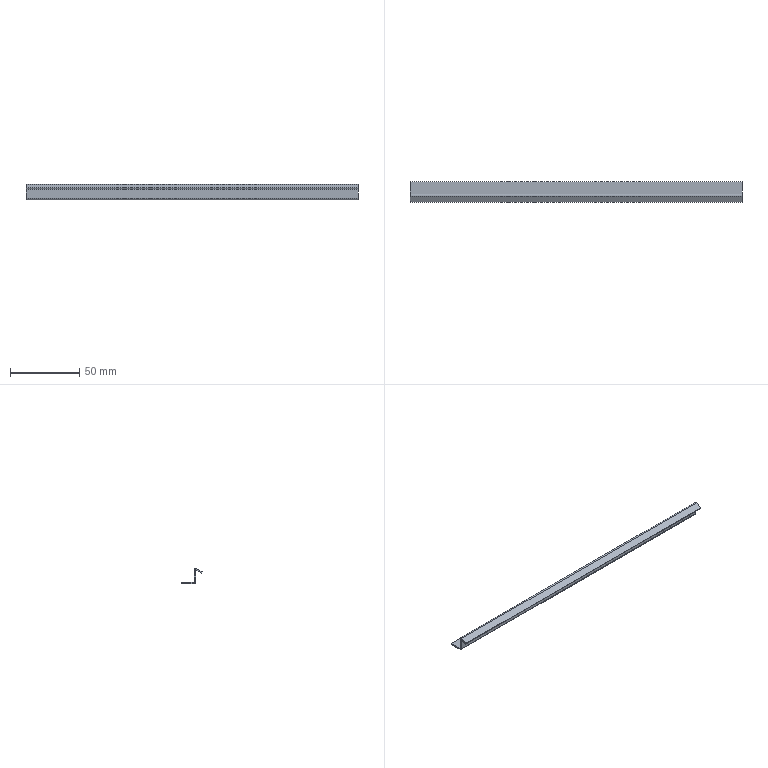Component | SolidWorks | Lampshade-1_Lampshade4-2 | 1 solid | 22 faces | box 240 x 14.83 x 10.93 mm | volume 5917 mm3 | plane 18 | cylinder 4 | commonest cylinder face diameters 2.2 x2 0.2 x2
STEP:
#1=COLOUR_RGB('',0.7922,0.8196,0.9333);
#2=FILL_AREA_STYLE_COLOUR('',#1);
#3=FILL_AREA_STYLE('',(#2));
#4=SURFACE_STYLE_FILL_AREA(#3);
#5=SURFACE_SIDE_STYLE('',(#4));
#6=SURFACE_STYLE_USAGE(.BOTH.,#5);
#7=PRESENTATION_STYLE_ASSIGNMENT((#6));
#8=CARTESIAN_POINT('',(-6.077,-0.7475,2.165));
#9=VERTEX_POINT('',#8);
#10=CARTESIAN_POINT('',(-6.077,-0.7475,2.205));
#11=VERTEX_POINT('',#10);
#12=CARTESIAN_POINT('',(-6.077,-0.7475,2.165));
#13=DIRECTION('',(-0.,0.,1.));
#14=VECTOR('',#13,39.37);
#15=LINE('',#12,#14);
#16=EDGE_CURVE('',#9,#11,#15,.T.);
#17=ORIENTED_EDGE('',*,*,#16,.F.);
#18=CARTESIAN_POINT('',(-6.077,-0.7908,2.209));
#19=VERTEX_POINT('',#18);
#20=CARTESIAN_POINT('',(-6.077,-0.7475,2.209));
#21=DIRECTION('',(-1.,0.,-0.));
#22=DIRECTION('',(0.,0.,-1.));
#23=AXIS2_PLACEMENT_3D('',#20,#21,#22);
#24=CIRCLE('',#23,0.04331);
#25=EDGE_CURVE('',#9,#19,#24,.T.);
#26=ORIENTED_EDGE('',*,*,#25,.T.);
#27=CARTESIAN_POINT('',(-6.077,-0.7514,2.209));
#28=VERTEX_POINT('',#27);
#29=CARTESIAN_POINT('',(-6.077,-0.7514,2.209));
#30=DIRECTION('',(-0.,-1.,0.));
#31=VECTOR('',#30,39.37);
#32=LINE('',#29,#31);
#33=EDGE_CURVE('',#28,#19,#32,.T.);
#34=ORIENTED_EDGE('',*,*,#33,.F.);
#35=CARTESIAN_POINT('',(-6.077,-0.7475,2.209));
#36=DIRECTION('',(-1.,0.,-0.));
#37=DIRECTION('',(0.,0.,1.));
#38=AXIS2_PLACEMENT_3D('',#35,#36,#37);
#39=CIRCLE('',#38,0.003937);
#40=EDGE_CURVE('',#11,#28,#39,.T.);
#41=ORIENTED_EDGE('',*,*,#40,.F.);
#42=EDGE_LOOP('',(#17,#26,#34,#41));
#43=FACE_OUTER_BOUND('',#42,.T.);
#44=CARTESIAN_POINT('',(-6.077,-0.7475,2.165));
#45=DIRECTION('',(-1.,0.,-0.));
#46=DIRECTION('',(-0.,0.,1.));
#47=AXIS2_PLACEMENT_3D('',#44,#45,#46);
#48=PLANE('',#47);
#49=ADVANCED_FACE('',(#43),#48,.T.);
#50=CARTESIAN_POINT('',(-6.077,-0.3971,2.165));
#51=VERTEX_POINT('',#50);
#52=CARTESIAN_POINT('',(-6.077,-0.3971,2.165));
#53=DIRECTION('',(-0.,-1.,0.));
#54=VECTOR('',#53,39.37);
#55=LINE('',#52,#54);
#56=EDGE_CURVE('',#51,#9,#55,.T.);
#57=ORIENTED_EDGE('',*,*,#56,.T.);
#58=ORIENTED_EDGE('',*,*,#16,.T.);
#59=CARTESIAN_POINT('',(-6.077,-0.3971,2.205));
#60=VERTEX_POINT('',#59);
#61=CARTESIAN_POINT('',(-6.077,-0.3971,2.205));
#62=DIRECTION('',(-0.,-1.,0.));
#63=VECTOR('',#62,39.37);
#64=LINE('',#61,#63);
#65=EDGE_CURVE('',#60,#11,#64,.T.);
#66=ORIENTED_EDGE('',*,*,#65,.F.);
#67=CARTESIAN_POINT('',(-6.077,-0.3971,2.165));
#68=DIRECTION('',(-0.,0.,1.));
#69=VECTOR('',#68,39.37);
#70=LINE('',#67,#69);
#71=EDGE_CURVE('',#51,#60,#70,.T.);
#72=ORIENTED_EDGE('',*,*,#71,.F.);
#73=EDGE_LOOP('',(#57,#58,#66,#72));
#74=FACE_OUTER_BOUND('',#73,.T.);
#75=CARTESIAN_POINT('',(-6.077,-0.7514,2.209));
#76=DIRECTION('',(-1.,0.,-0.));
#77=DIRECTION('',(-0.,0.,1.));
#78=AXIS2_PLACEMENT_3D('',#75,#76,#77);
#79=PLANE('',#78);
#80=ADVANCED_FACE('',(#74),#79,.T.);
#81=CARTESIAN_POINT('',(3.372,-0.7908,2.209));
#82=VERTEX_POINT('',#81);
#83=CARTESIAN_POINT('',(3.372,-0.7514,2.209));
#84=VERTEX_POINT('',#83);
#85=CARTESIAN_POINT('',(3.372,-0.7908,2.209));
#86=DIRECTION('',(0.,1.,-0.));
#87=VECTOR('',#86,39.37);
#88=LINE('',#85,#87);
#89=EDGE_CURVE('',#82,#84,#88,.T.);
#90=ORIENTED_EDGE('',*,*,#89,.F.);
#91=CARTESIAN_POINT('',(3.372,-0.7475,2.165));
#92=VERTEX_POINT('',#91);
#93=CARTESIAN_POINT('',(3.372,-0.7475,2.209));
#94=DIRECTION('',(-1.,0.,-0.));
#95=DIRECTION('',(0.,0.,-1.));
#96=AXIS2_PLACEMENT_3D('',#93,#94,#95);
#97=CIRCLE('',#96,0.04331);
#98=EDGE_CURVE('',#92,#82,#97,.T.);
#99=ORIENTED_EDGE('',*,*,#98,.F.);
#100=CARTESIAN_POINT('',(3.372,-0.7475,2.205));
#101=VERTEX_POINT('',#100);
#102=CARTESIAN_POINT('',(3.372,-0.7475,2.205));
#103=DIRECTION('',(0.,-0.,-1.));
#104=VECTOR('',#103,39.37);
#105=LINE('',#102,#104);
#106=EDGE_CURVE('',#101,#92,#105,.T.);
#107=ORIENTED_EDGE('',*,*,#106,.F.);
#108=CARTESIAN_POINT('',(3.372,-0.7475,2.209));
#109=DIRECTION('',(-1.,0.,-0.));
#110=DIRECTION('',(0.,0.,1.));
#111=AXIS2_PLACEMENT_3D('',#108,#109,#110);
#112=CIRCLE('',#111,0.003937);
#113=EDGE_CURVE('',#101,#84,#112,.T.);
#114=ORIENTED_EDGE('',*,*,#113,.T.);
#115=EDGE_LOOP('',(#90,#99,#107,#114));
#116=FACE_OUTER_BOUND('',#115,.T.);
#117=CARTESIAN_POINT('',(3.372,-0.7908,2.209));
#118=DIRECTION('',(1.,-0.,0.));
#119=DIRECTION('',(0.,-0.,-1.));
#120=AXIS2_PLACEMENT_3D('',#117,#118,#119);
#121=PLANE('',#120);
#122=ADVANCED_FACE('',(#116),#121,.T.);
#123=CARTESIAN_POINT('',(3.372,-0.7908,2.552));
#124=VERTEX_POINT('',#123);
#125=CARTESIAN_POINT('',(3.372,-0.7908,2.165));
#126=DIRECTION('',(-0.,0.,1.));
#127=VECTOR('',#126,39.37);
#128=LINE('',#125,#127);
#129=EDGE_CURVE('',#82,#124,#128,.T.);
#130=ORIENTED_EDGE('',*,*,#129,.F.);
#131=ORIENTED_EDGE('',*,*,#89,.T.);
#132=CARTESIAN_POINT('',(3.372,-0.7514,2.552));
#133=VERTEX_POINT('',#132);
#134=CARTESIAN_POINT('',(3.372,-0.7514,2.165));
#135=DIRECTION('',(-0.,0.,1.));
#136=VECTOR('',#135,39.37);
#137=LINE('',#134,#136);
#138=EDGE_CURVE('',#84,#133,#137,.T.);
#139=ORIENTED_EDGE('',*,*,#138,.T.);
#140=CARTESIAN_POINT('',(3.372,-0.7514,2.552));
#141=DIRECTION('',(-0.,-1.,0.));
#142=VECTOR('',#141,39.37);
#143=LINE('',#140,#142);
#144=EDGE_CURVE('',#133,#124,#143,.T.);
#145=ORIENTED_EDGE('',*,*,#144,.T.);
#146=EDGE_LOOP('',(#130,#131,#139,#145));
#147=FACE_OUTER_BOUND('',#146,.T.);
#148=CARTESIAN_POINT('',(3.372,-0.7475,2.205));
#149=DIRECTION('',(1.,-0.,0.));
#150=DIRECTION('',(0.,-0.,-1.));
#151=AXIS2_PLACEMENT_3D('',#148,#149,#150);
#152=PLANE('',#151);
#153=ADVANCED_FACE('',(#147),#152,.T.);
#154=CARTESIAN_POINT('',(-6.077,-0.7908,2.552));
#155=VERTEX_POINT('',#154);
#156=CARTESIAN_POINT('',(-6.077,-0.7514,2.552));
#157=VERTEX_POINT('',#156);
#158=CARTESIAN_POINT('',(-6.077,-0.7908,2.552));
#159=DIRECTION('',(0.,1.,-0.));
#160=VECTOR('',#159,39.37);
#161=LINE('',#158,#160);
#162=EDGE_CURVE('',#155,#157,#161,.T.);
#163=ORIENTED_EDGE('',*,*,#162,.F.);
#164=CARTESIAN_POINT('',(-6.077,-0.7967,2.556));
#165=VERTEX_POINT('',#164);
#166=CARTESIAN_POINT('',(-6.077,-0.7948,2.552));
#167=DIRECTION('',(1.,-0.,0.));
#168=DIRECTION('',(0.,0.,1.));
#169=AXIS2_PLACEMENT_3D('',#166,#167,#168);
#170=CIRCLE('',#169,0.003937);
#171=EDGE_CURVE('',#155,#165,#170,.T.);
#172=ORIENTED_EDGE('',*,*,#171,.T.);
#173=CARTESIAN_POINT('',(-6.077,-0.8164,2.59));
#174=VERTEX_POINT('',#173);
#175=CARTESIAN_POINT('',(-6.077,-0.8164,2.59));
#176=DIRECTION('',(0.,0.5,-0.866));
#177=VECTOR('',#176,39.37);
#178=LINE('',#175,#177);
#179=EDGE_CURVE('',#174,#165,#178,.T.);
#180=ORIENTED_EDGE('',*,*,#179,.F.);
#181=CARTESIAN_POINT('',(-6.077,-0.7948,2.552));
#182=DIRECTION('',(1.,-0.,0.));
#183=DIRECTION('',(0.,0.,1.));
#184=AXIS2_PLACEMENT_3D('',#181,#182,#183);
#185=CIRCLE('',#184,0.04331);
#186=EDGE_CURVE('',#157,#174,#185,.T.);
#187=ORIENTED_EDGE('',*,*,#186,.F.);
#188=EDGE_LOOP('',(#163,#172,#180,#187));
#189=FACE_OUTER_BOUND('',#188,.T.);
#190=CARTESIAN_POINT('',(-6.077,-0.7908,2.552));
#191=DIRECTION('',(-1.,0.,-0.));
#192=DIRECTION('',(-0.,0.,1.));
#193=AXIS2_PLACEMENT_3D('',#190,#191,#192);
#194=PLANE('',#193);
#195=ADVANCED_FACE('',(#189),#194,.T.);
#196=CARTESIAN_POINT('',(-6.077,-0.7908,2.165));
#197=DIRECTION('',(-0.,0.,1.));
#198=VECTOR('',#197,39.37);
#199=LINE('',#196,#198);
#200=EDGE_CURVE('',#19,#155,#199,.T.);
#201=ORIENTED_EDGE('',*,*,#200,.T.);
#202=ORIENTED_EDGE('',*,*,#162,.T.);
#203=CARTESIAN_POINT('',(-6.077,-0.7514,2.165));
#204=DIRECTION('',(-0.,0.,1.));
#205=VECTOR('',#204,39.37);
#206=LINE('',#203,#205);
#207=EDGE_CURVE('',#28,#157,#206,.T.);
#208=ORIENTED_EDGE('',*,*,#207,.F.);
#209=ORIENTED_EDGE('',*,*,#33,.T.);
#210=EDGE_LOOP('',(#201,#202,#208,#209));
#211=FACE_OUTER_BOUND('',#210,.T.);
#212=CARTESIAN_POINT('',(-6.077,-0.8164,2.59));
#213=DIRECTION('',(-1.,0.,-0.));
#214=DIRECTION('',(-0.,0.,1.));
#215=AXIS2_PLACEMENT_3D('',#212,#213,#214);
#216=PLANE('',#215);
#217=ADVANCED_FACE('',(#211),#216,.T.);
#218=CARTESIAN_POINT('',(3.372,-0.7967,2.556));
#219=VERTEX_POINT('',#218);
#220=CARTESIAN_POINT('',(3.372,-0.8164,2.59));
#221=VERTEX_POINT('',#220);
#222=CARTESIAN_POINT('',(3.372,-0.7967,2.556));
#223=DIRECTION('',(-0.,-0.5,0.866));
#224=VECTOR('',#223,39.37);
#225=LINE('',#222,#224);
#226=EDGE_CURVE('',#219,#221,#225,.T.);
#227=ORIENTED_EDGE('',*,*,#226,.F.);
#228=CARTESIAN_POINT('',(3.372,-0.7948,2.552));
#229=DIRECTION('',(1.,-0.,0.));
#230=DIRECTION('',(0.,0.,1.));
#231=AXIS2_PLACEMENT_3D('',#228,#229,#230);
#232=CIRCLE('',#231,0.003937);
#233=EDGE_CURVE('',#124,#219,#232,.T.);
#234=ORIENTED_EDGE('',*,*,#233,.F.);
#235=ORIENTED_EDGE('',*,*,#144,.F.);
#236=CARTESIAN_POINT('',(3.372,-0.7948,2.552));
#237=DIRECTION('',(1.,-0.,0.));
#238=DIRECTION('',(0.,0.,1.));
#239=AXIS2_PLACEMENT_3D('',#236,#237,#238);
#240=CIRCLE('',#239,0.04331);
#241=EDGE_CURVE('',#133,#221,#240,.T.);
#242=ORIENTED_EDGE('',*,*,#241,.T.);
#243=EDGE_LOOP('',(#227,#234,#235,#242));
#244=FACE_OUTER_BOUND('',#243,.T.);
#245=CARTESIAN_POINT('',(3.372,-0.7967,2.556));
#246=DIRECTION('',(1.,-0.,0.));
#247=DIRECTION('',(0.,-0.,-1.));
#248=AXIS2_PLACEMENT_3D('',#245,#246,#247);
#249=PLANE('',#248);
#250=ADVANCED_FACE('',(#244),#249,.T.);
#251=CARTESIAN_POINT('',(3.372,-0.9613,2.461));
#252=VERTEX_POINT('',#251);
#253=CARTESIAN_POINT('',(3.372,-0.7908,2.559));
#254=DIRECTION('',(-0.,-0.866,-0.5));
#255=VECTOR('',#254,39.37);
#256=LINE('',#253,#255);
#257=EDGE_CURVE('',#219,#252,#256,.T.);
#258=ORIENTED_EDGE('',*,*,#257,.F.);
#259=ORIENTED_EDGE('',*,*,#226,.T.);
#260=CARTESIAN_POINT('',(3.372,-0.981,2.495));
#261=VERTEX_POINT('',#260);
#262=CARTESIAN_POINT('',(3.372,-0.8105,2.593));
#263=DIRECTION('',(-0.,-0.866,-0.5));
#264=VECTOR('',#263,39.37);
#265=LINE('',#262,#264);
#266=EDGE_CURVE('',#221,#261,#265,.T.);
#267=ORIENTED_EDGE('',*,*,#266,.T.);
#268=CARTESIAN_POINT('',(3.372,-0.981,2.495));
#269=DIRECTION('',(0.,0.5,-0.866));
#270=VECTOR('',#269,39.37);
#271=LINE('',#268,#270);
#272=EDGE_CURVE('',#261,#252,#271,.T.);
#273=ORIENTED_EDGE('',*,*,#272,.T.);
#274=EDGE_LOOP('',(#258,#259,#267,#273));
#275=FACE_OUTER_BOUND('',#274,.T.);
#276=CARTESIAN_POINT('',(3.372,-0.7514,2.552));
#277=DIRECTION('',(1.,-0.,0.));
#278=DIRECTION('',(0.,-0.,-1.));
#279=AXIS2_PLACEMENT_3D('',#276,#277,#278);
#280=PLANE('',#279);
#281=ADVANCED_FACE('',(#275),#280,.T.);
#282=ORIENTED_EDGE('',*,*,#257,.T.);
#283=CARTESIAN_POINT('',(-6.077,-0.9613,2.461));
#284=VERTEX_POINT('',#283);
#285=CARTESIAN_POINT('',(-6.077,-0.9613,2.461));
#286=DIRECTION('',(1.,-0.,0.));
#287=VECTOR('',#286,39.37);
#288=LINE('',#285,#287);
#289=EDGE_CURVE('',#284,#252,#288,.T.);
#290=ORIENTED_EDGE('',*,*,#289,.F.);
#291=CARTESIAN_POINT('',(-6.077,-0.7908,2.559));
#292=DIRECTION('',(-0.,-0.866,-0.5));
#293=VECTOR('',#292,39.37);
#294=LINE('',#291,#293);
#295=EDGE_CURVE('',#165,#284,#294,.T.);
#296=ORIENTED_EDGE('',*,*,#295,.F.);
#297=CARTESIAN_POINT('',(-6.077,-0.7967,2.556));
#298=DIRECTION('',(1.,-0.,0.));
#299=VECTOR('',#298,39.37);
#300=LINE('',#297,#299);
#301=EDGE_CURVE('',#165,#219,#300,.T.);
#302=ORIENTED_EDGE('',*,*,#301,.T.);
#303=EDGE_LOOP('',(#282,#290,#296,#302));
#304=FACE_OUTER_BOUND('',#303,.T.);
#305=CARTESIAN_POINT('',(-6.077,-0.7908,2.559));
#306=DIRECTION('',(-0.,-0.5,0.866));
#307=DIRECTION('',(0.,0.866,0.5));
#308=AXIS2_PLACEMENT_3D('',#305,#306,#307);
#309=PLANE('',#308);
#310=ADVANCED_FACE('',(#304),#309,.F.);
#311=ORIENTED_EDGE('',*,*,#272,.F.);
#312=CARTESIAN_POINT('',(-6.077,-0.981,2.495));
#313=VERTEX_POINT('',#312);
#314=CARTESIAN_POINT('',(-6.077,-0.981,2.495));
#315=DIRECTION('',(1.,-0.,0.));
#316=VECTOR('',#315,39.37);
#317=LINE('',#314,#316);
#318=EDGE_CURVE('',#313,#261,#317,.T.);
#319=ORIENTED_EDGE('',*,*,#318,.F.);
#320=CARTESIAN_POINT('',(-6.077,-0.981,2.495));
#321=DIRECTION('',(0.,0.5,-0.866));
#322=VECTOR('',#321,39.37);
#323=LINE('',#320,#322);
#324=EDGE_CURVE('',#313,#284,#323,.T.);
#325=ORIENTED_EDGE('',*,*,#324,.T.);
#326=ORIENTED_EDGE('',*,*,#289,.T.);
#327=EDGE_LOOP('',(#311,#319,#325,#326));
#328=FACE_OUTER_BOUND('',#327,.T.);
#329=CARTESIAN_POINT('',(-6.077,-0.981,2.495));
#330=DIRECTION('',(-0.,-0.866,-0.5));
#331=DIRECTION('',(-0.,-0.5,0.866));
#332=AXIS2_PLACEMENT_3D('',#329,#330,#331);
#333=PLANE('',#332);
#334=ADVANCED_FACE('',(#328),#333,.T.);
#335=ORIENTED_EDGE('',*,*,#266,.F.);
#336=CARTESIAN_POINT('',(-6.077,-0.8164,2.59));
#337=DIRECTION('',(1.,-0.,0.));
#338=VECTOR('',#337,39.37);
#339=LINE('',#336,#338);
#340=EDGE_CURVE('',#174,#221,#339,.T.);
#341=ORIENTED_EDGE('',*,*,#340,.F.);
#342=CARTESIAN_POINT('',(-6.077,-0.8105,2.593));
#343=DIRECTION('',(-0.,-0.866,-0.5));
#344=VECTOR('',#343,39.37);
#345=LINE('',#342,#344);
#346=EDGE_CURVE('',#174,#313,#345,.T.);
#347=ORIENTED_EDGE('',*,*,#346,.T.);
#348=ORIENTED_EDGE('',*,*,#318,.T.);
#349=EDGE_LOOP('',(#335,#341,#347,#348));
#350=FACE_OUTER_BOUND('',#349,.T.);
#351=CARTESIAN_POINT('',(-6.077,-0.8105,2.593));
#352=DIRECTION('',(-0.,-0.5,0.866));
#353=DIRECTION('',(0.,0.866,0.5));
#354=AXIS2_PLACEMENT_3D('',#351,#352,#353);
#355=PLANE('',#354);
#356=ADVANCED_FACE('',(#350),#355,.T.);
#357=ORIENTED_EDGE('',*,*,#241,.F.);
#358=CARTESIAN_POINT('',(-6.077,-0.7514,2.552));
#359=DIRECTION('',(1.,-0.,0.));
#360=VECTOR('',#359,39.37);
#361=LINE('',#358,#360);
#362=EDGE_CURVE('',#157,#133,#361,.T.);
#363=ORIENTED_EDGE('',*,*,#362,.F.);
#364=ORIENTED_EDGE('',*,*,#186,.T.);
#365=ORIENTED_EDGE('',*,*,#340,.T.);
#366=EDGE_LOOP('',(#357,#363,#364,#365));
#367=FACE_OUTER_BOUND('',#366,.T.);
#368=CARTESIAN_POINT('',(-6.077,-0.7948,2.552));
#369=DIRECTION('',(1.,-0.,0.));
#370=DIRECTION('',(0.,0.,-1.));
#371=AXIS2_PLACEMENT_3D('',#368,#369,#370);
#372=CYLINDRICAL_SURFACE('',#371,0.04331);
#373=ADVANCED_FACE('',(#367),#372,.T.);
#374=ORIENTED_EDGE('',*,*,#138,.F.);
#375=CARTESIAN_POINT('',(-6.077,-0.7514,2.209));
#376=DIRECTION('',(1.,-0.,0.));
#377=VECTOR('',#376,39.37);
#378=LINE('',#375,#377);
#379=EDGE_CURVE('',#28,#84,#378,.T.);
#380=ORIENTED_EDGE('',*,*,#379,.F.);
#381=ORIENTED_EDGE('',*,*,#207,.T.);
#382=ORIENTED_EDGE('',*,*,#362,.T.);
#383=EDGE_LOOP('',(#374,#380,#381,#382));
#384=FACE_OUTER_BOUND('',#383,.T.);
#385=CARTESIAN_POINT('',(-6.077,-0.7514,2.165));
#386=DIRECTION('',(0.,1.,-0.));
#387=DIRECTION('',(-1.,0.,-0.));
#388=AXIS2_PLACEMENT_3D('',#385,#386,#387);
#389=PLANE('',#388);
#390=ADVANCED_FACE('',(#384),#389,.T.);
#391=ORIENTED_EDGE('',*,*,#113,.F.);
#392=CARTESIAN_POINT('',(-6.077,-0.7475,2.205));
#393=DIRECTION('',(1.,-0.,0.));
#394=VECTOR('',#393,39.37);
#395=LINE('',#392,#394);
#396=EDGE_CURVE('',#11,#101,#395,.T.);
#397=ORIENTED_EDGE('',*,*,#396,.F.);
#398=ORIENTED_EDGE('',*,*,#40,.T.);
#399=ORIENTED_EDGE('',*,*,#379,.T.);
#400=EDGE_LOOP('',(#391,#397,#398,#399));
#401=FACE_OUTER_BOUND('',#400,.T.);
#402=CARTESIAN_POINT('',(-6.077,-0.7475,2.209));
#403=DIRECTION('',(1.,-0.,0.));
#404=DIRECTION('',(0.,0.,-1.));
#405=AXIS2_PLACEMENT_3D('',#402,#403,#404);
#406=CYLINDRICAL_SURFACE('',#405,0.003937);
#407=ADVANCED_FACE('',(#401),#406,.F.);
#408=CARTESIAN_POINT('',(3.372,-0.3971,2.205));
#409=VERTEX_POINT('',#408);
#410=CARTESIAN_POINT('',(3.372,-0.3971,2.205));
#411=DIRECTION('',(-0.,-1.,0.));
#412=VECTOR('',#411,39.37);
#413=LINE('',#410,#412);
#414=EDGE_CURVE('',#409,#101,#413,.T.);
#415=ORIENTED_EDGE('',*,*,#414,.F.);
#416=CARTESIAN_POINT('',(-6.077,-0.3971,2.205));
#417=DIRECTION('',(1.,-0.,0.));
#418=VECTOR('',#417,39.37);
#419=LINE('',#416,#418);
#420=EDGE_CURVE('',#60,#409,#419,.T.);
#421=ORIENTED_EDGE('',*,*,#420,.F.);
#422=ORIENTED_EDGE('',*,*,#65,.T.);
#423=ORIENTED_EDGE('',*,*,#396,.T.);
#424=EDGE_LOOP('',(#415,#421,#422,#423));
#425=FACE_OUTER_BOUND('',#424,.T.);
#426=CARTESIAN_POINT('',(-6.077,-0.3971,2.205));
#427=DIRECTION('',(-0.,0.,1.));
#428=DIRECTION('',(1.,-0.,0.));
#429=AXIS2_PLACEMENT_3D('',#426,#427,#428);
#430=PLANE('',#429);
#431=ADVANCED_FACE('',(#425),#430,.T.);
#432=CARTESIAN_POINT('',(3.372,-0.3971,2.165));
#433=VERTEX_POINT('',#432);
#434=CARTESIAN_POINT('',(3.372,-0.3971,2.165));
#435=DIRECTION('',(-0.,0.,1.));
#436=VECTOR('',#435,39.37);
#437=LINE('',#434,#436);
#438=EDGE_CURVE('',#433,#409,#437,.T.);
#439=ORIENTED_EDGE('',*,*,#438,.F.);
#440=CARTESIAN_POINT('',(-6.077,-0.3971,2.165));
#441=DIRECTION('',(1.,-0.,0.));
#442=VECTOR('',#441,39.37);
#443=LINE('',#440,#442);
#444=EDGE_CURVE('',#51,#433,#443,.T.);
#445=ORIENTED_EDGE('',*,*,#444,.F.);
#446=ORIENTED_EDGE('',*,*,#71,.T.);
#447=ORIENTED_EDGE('',*,*,#420,.T.);
#448=EDGE_LOOP('',(#439,#445,#446,#447));
#449=FACE_OUTER_BOUND('',#448,.T.);
#450=CARTESIAN_POINT('',(-6.077,-0.3971,2.165));
#451=DIRECTION('',(0.,1.,-0.));
#452=DIRECTION('',(-1.,0.,-0.));
#453=AXIS2_PLACEMENT_3D('',#450,#451,#452);
#454=PLANE('',#453);
#455=ADVANCED_FACE('',(#449),#454,.T.);
#456=CARTESIAN_POINT('',(3.372,-0.3971,2.165));
#457=DIRECTION('',(-0.,-1.,0.));
#458=VECTOR('',#457,39.37);
#459=LINE('',#456,#458);
#460=EDGE_CURVE('',#433,#92,#459,.T.);
#461=ORIENTED_EDGE('',*,*,#460,.T.);
#462=CARTESIAN_POINT('',(-6.077,-0.7475,2.165));
#463=DIRECTION('',(1.,-0.,0.));
#464=VECTOR('',#463,39.37);
#465=LINE('',#462,#464);
#466=EDGE_CURVE('',#9,#92,#465,.T.);
#467=ORIENTED_EDGE('',*,*,#466,.F.);
#468=ORIENTED_EDGE('',*,*,#56,.F.);
#469=ORIENTED_EDGE('',*,*,#444,.T.);
#470=EDGE_LOOP('',(#461,#467,#468,#469));
#471=FACE_OUTER_BOUND('',#470,.T.);
#472=CARTESIAN_POINT('',(-6.077,-0.3971,2.165));
#473=DIRECTION('',(-0.,0.,1.));
#474=DIRECTION('',(1.,-0.,0.));
#475=AXIS2_PLACEMENT_3D('',#472,#473,#474);
#476=PLANE('',#475);
#477=ADVANCED_FACE('',(#471),#476,.F.);
#478=ORIENTED_EDGE('',*,*,#98,.T.);
#479=CARTESIAN_POINT('',(-6.077,-0.7908,2.209));
#480=DIRECTION('',(1.,-0.,0.));
#481=VECTOR('',#480,39.37);
#482=LINE('',#479,#481);
#483=EDGE_CURVE('',#19,#82,#482,.T.);
#484=ORIENTED_EDGE('',*,*,#483,.F.);
#485=ORIENTED_EDGE('',*,*,#25,.F.);
#486=ORIENTED_EDGE('',*,*,#466,.T.);
#487=EDGE_LOOP('',(#478,#484,#485,#486));
#488=FACE_OUTER_BOUND('',#487,.T.);
#489=CARTESIAN_POINT('',(-6.077,-0.7475,2.209));
#490=DIRECTION('',(1.,-0.,0.));
#491=DIRECTION('',(0.,0.,-1.));
#492=AXIS2_PLACEMENT_3D('',#489,#490,#491);
#493=CYLINDRICAL_SURFACE('',#492,0.04331);
#494=ADVANCED_FACE('',(#488),#493,.T.);
#495=ORIENTED_EDGE('',*,*,#129,.T.);
#496=CARTESIAN_POINT('',(-6.077,-0.7908,2.552));
#497=DIRECTION('',(1.,-0.,0.));
#498=VECTOR('',#497,39.37);
#499=LINE('',#496,#498);
#500=EDGE_CURVE('',#155,#124,#499,.T.);
#501=ORIENTED_EDGE('',*,*,#500,.F.);
#502=ORIENTED_EDGE('',*,*,#200,.F.);
#503=ORIENTED_EDGE('',*,*,#483,.T.);
#504=EDGE_LOOP('',(#495,#501,#502,#503));
#505=FACE_OUTER_BOUND('',#504,.T.);
#506=CARTESIAN_POINT('',(-6.077,-0.7908,2.165));
#507=DIRECTION('',(0.,1.,-0.));
#508=DIRECTION('',(-1.,0.,-0.));
#509=AXIS2_PLACEMENT_3D('',#506,#507,#508);
#510=PLANE('',#509);
#511=ADVANCED_FACE('',(#505),#510,.F.);
#512=ORIENTED_EDGE('',*,*,#233,.T.);
#513=ORIENTED_EDGE('',*,*,#301,.F.);
#514=ORIENTED_EDGE('',*,*,#171,.F.);
#515=ORIENTED_EDGE('',*,*,#500,.T.);
#516=EDGE_LOOP('',(#512,#513,#514,#515));
#517=FACE_OUTER_BOUND('',#516,.T.);
#518=CARTESIAN_POINT('',(-6.077,-0.7948,2.552));
#519=DIRECTION('',(1.,-0.,0.));
#520=DIRECTION('',(0.,0.,-1.));
#521=AXIS2_PLACEMENT_3D('',#518,#519,#520);
#522=CYLINDRICAL_SURFACE('',#521,0.003937);
#523=ADVANCED_FACE('',(#517),#522,.F.);
#524=ORIENTED_EDGE('',*,*,#295,.T.);
#525=ORIENTED_EDGE('',*,*,#324,.F.);
#526=ORIENTED_EDGE('',*,*,#346,.F.);
#527=ORIENTED_EDGE('',*,*,#179,.T.);
#528=EDGE_LOOP('',(#524,#525,#526,#527));
#529=FACE_OUTER_BOUND('',#528,.T.);
#530=CARTESIAN_POINT('',(-6.077,-0.7948,2.552));
#531=DIRECTION('',(-1.,0.,-0.));
#532=DIRECTION('',(-0.,0.,1.));
#533=AXIS2_PLACEMENT_3D('',#530,#531,#532);
#534=PLANE('',#533);
#535=ADVANCED_FACE('',(#529),#534,.T.);
#536=ORIENTED_EDGE('',*,*,#414,.T.);
#537=ORIENTED_EDGE('',*,*,#106,.T.);
#538=ORIENTED_EDGE('',*,*,#460,.F.);
#539=ORIENTED_EDGE('',*,*,#438,.T.);
#540=EDGE_LOOP('',(#536,#537,#538,#539));
#541=FACE_OUTER_BOUND('',#540,.T.);
#542=CARTESIAN_POINT('',(3.372,-0.7948,2.552));
#543=DIRECTION('',(-1.,0.,-0.));
#544=DIRECTION('',(-0.,0.,1.));
#545=AXIS2_PLACEMENT_3D('',#542,#543,#544);
#546=PLANE('',#545);
#547=ADVANCED_FACE('',(#541),#546,.F.);
#548=CLOSED_SHELL('',(#49,#80,#122,#153,#195,#217,#250,#281,#310,#334,#356,#373,#390,#407,#431,#455,#477,#494,#511,#523,#535,#547));
#549=MANIFOLD_SOLID_BREP('',#548);
#550=STYLED_ITEM('',(#7),#549);
#551=(LENGTH_UNIT()NAMED_UNIT(*)SI_UNIT($,.METRE.));
#552=LENGTH_MEASURE_WITH_UNIT(LENGTH_MEASURE(0.0254),#551);
#553=DIMENSIONAL_EXPONENTS(1.,0.,0.,0.,0.,0.,0.);
#554=(CONVERSION_BASED_UNIT('',#552)LENGTH_UNIT()NAMED_UNIT(#553));
#555=UNCERTAINTY_MEASURE_WITH_UNIT(LENGTH_MEASURE(0.00001),#554,'','');
#556=(NAMED_UNIT(*)PLANE_ANGLE_UNIT()SI_UNIT($,.RADIAN.));
#557=(NAMED_UNIT(*)SI_UNIT($,.STERADIAN.)SOLID_ANGLE_UNIT());
#558=(GEOMETRIC_REPRESENTATION_CONTEXT(3)GLOBAL_UNCERTAINTY_ASSIGNED_CONTEXT((#555))GLOBAL_UNIT_ASSIGNED_CONTEXT((#554,#556,#557))REPRESENTATION_CONTEXT('',''));
#559=MECHANICAL_DESIGN_GEOMETRIC_PRESENTATION_REPRESENTATION('',(#550),#558);
#560=CARTESIAN_POINT('',(0.,0.,0.));
#561=DIRECTION('',(0.,0.,1.));
#562=DIRECTION('',(1.,0.,0.));
#563=AXIS2_PLACEMENT_3D('',#560,#561,#562);
#564=(LENGTH_UNIT()NAMED_UNIT(*)SI_UNIT($,.METRE.));
#565=LENGTH_MEASURE_WITH_UNIT(LENGTH_MEASURE(0.0254),#564);
#566=DIMENSIONAL_EXPONENTS(1.,0.,0.,0.,0.,0.,0.);
#567=(CONVERSION_BASED_UNIT('',#565)LENGTH_UNIT()NAMED_UNIT(#566));
#568=UNCERTAINTY_MEASURE_WITH_UNIT(LENGTH_MEASURE(0.00001),#567,'','');
#569=(NAMED_UNIT(*)PLANE_ANGLE_UNIT()SI_UNIT($,.RADIAN.));
#570=(NAMED_UNIT(*)SI_UNIT($,.STERADIAN.)SOLID_ANGLE_UNIT());
#571=(GEOMETRIC_REPRESENTATION_CONTEXT(3)GLOBAL_UNCERTAINTY_ASSIGNED_CONTEXT((#568))GLOBAL_UNIT_ASSIGNED_CONTEXT((#567,#569,#570))REPRESENTATION_CONTEXT('',''));
#572=ADVANCED_BREP_SHAPE_REPRESENTATION('',(#549,#563),#571);
#573=PRESENTATION_LAYER_ASSIGNMENT('','',(#550));